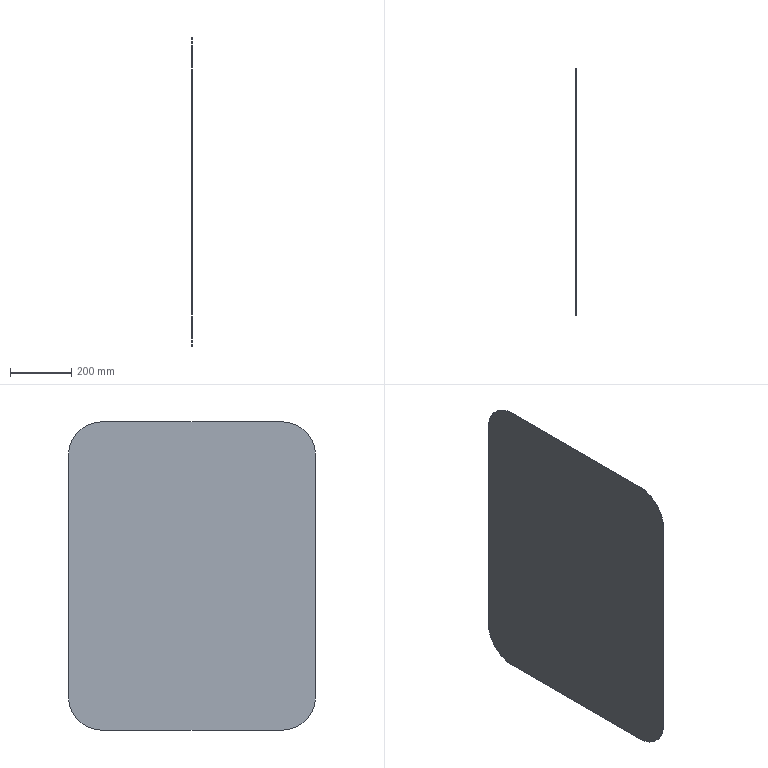Component | NX | CB2_1 | 1 solid | 10 faces | volume 1209123 mm3 | plane 6 | cylinder 4 | commonest cylinder face diameters 218 x4